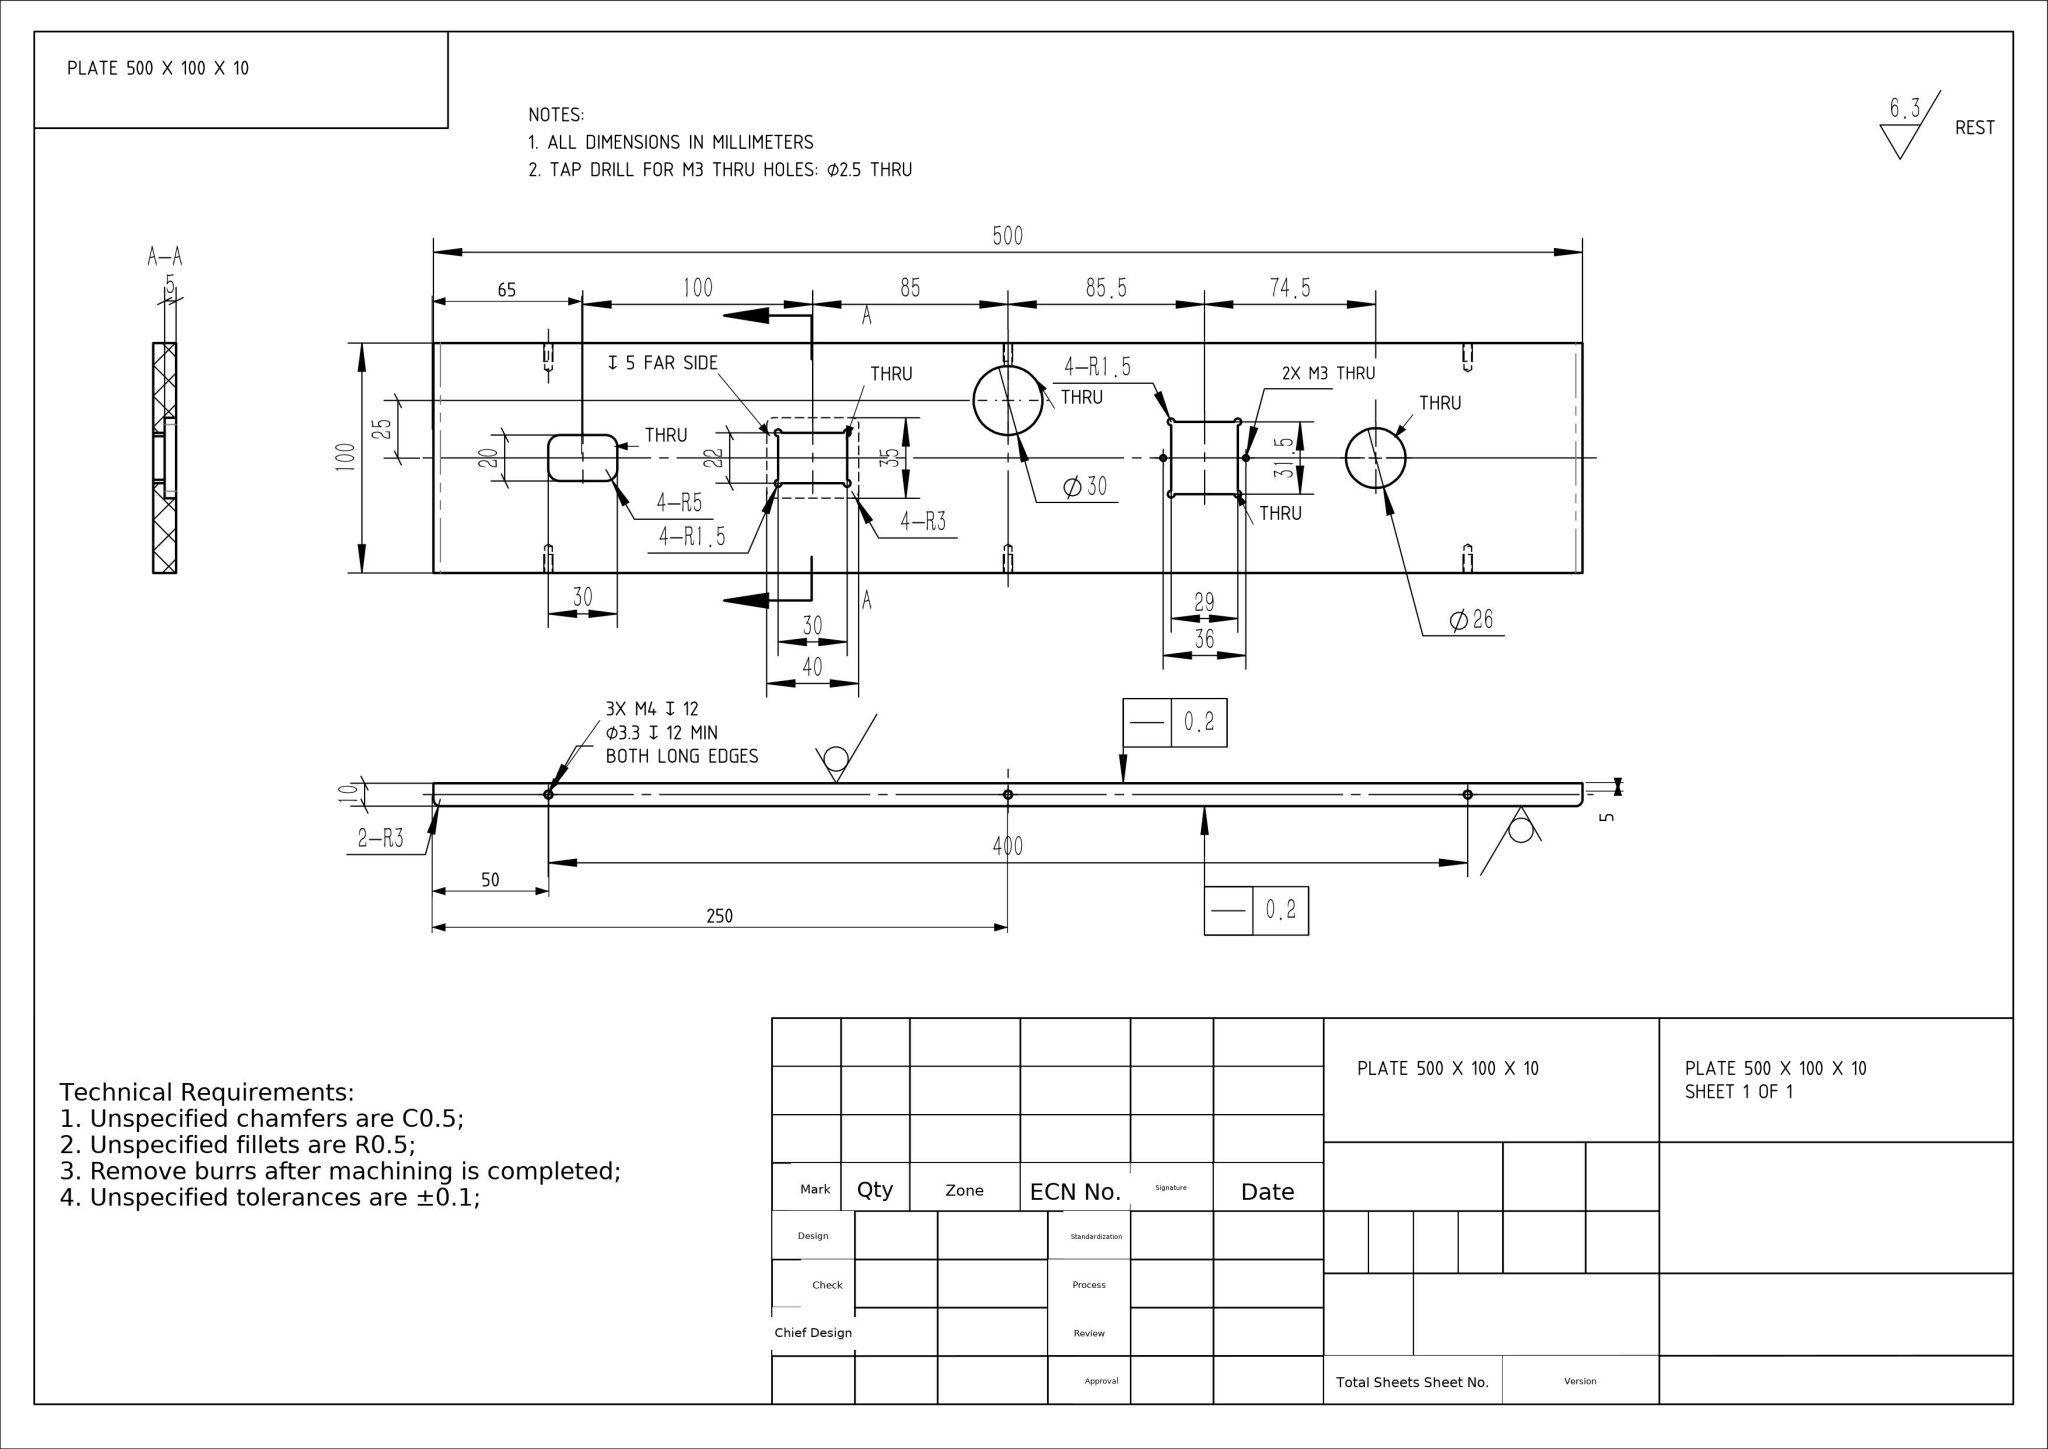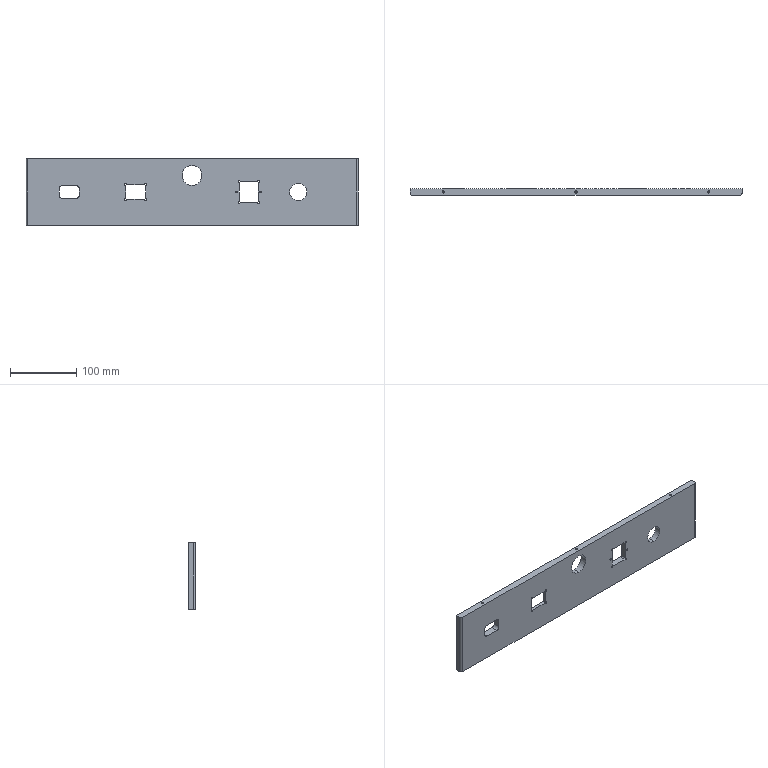Part | NX | mm | 1 solid | 75 faces | box 500 x 10 x 100 mm | volume 461046 mm3 | cylinder 42 | plane 23 | cone 10 | commonest cylinder face diameters 3 x12 3.3 x12 6 x6 2.5 x4 10 x4 30 x2 26 x2